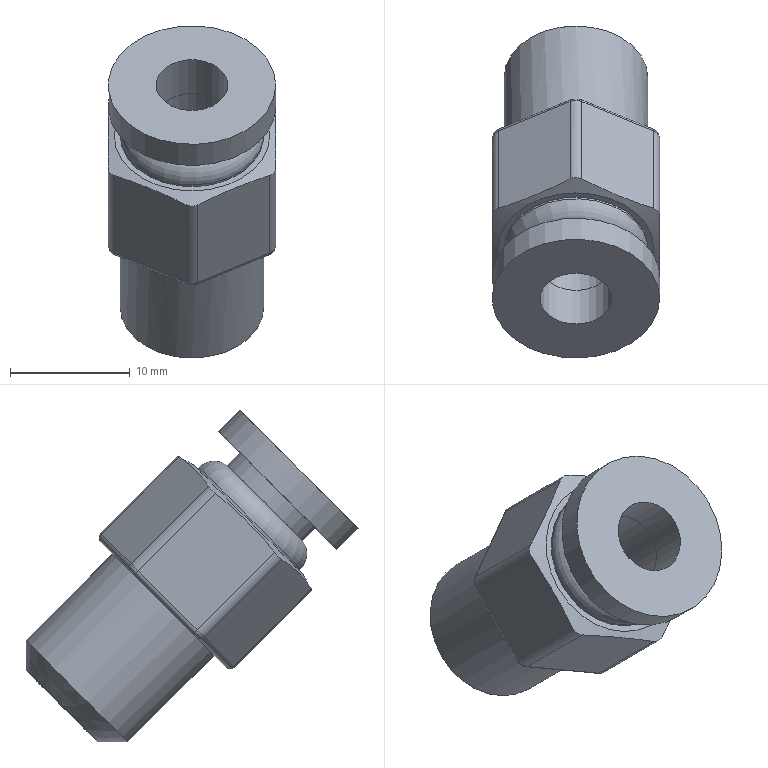Component | NX | AIR_PIPE_CONNECTOR_2 | 2 solids | 40 faces | volume 2882 mm3 | cylinder 18 | plane 13 | spline 6 | cone 2 | torus 1 | commonest cylinder face diameters 2 x6 1 x6 12 x2 6 x2 14 x1 9 x1